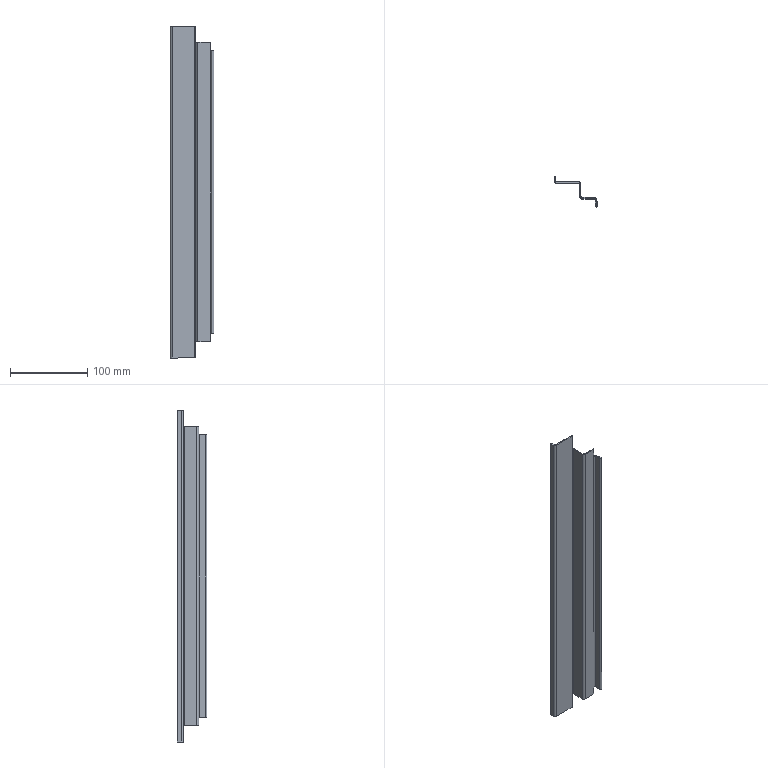Component | SolidWorks | SmallDoorFrameTwo100-4 | 1 solid | 54 faces | volume 56833 mm3 | plane 44 | cylinder 10 | commonest cylinder face diameters 2.4 x4 5.4 x4 3.1 x1 0.1 x1